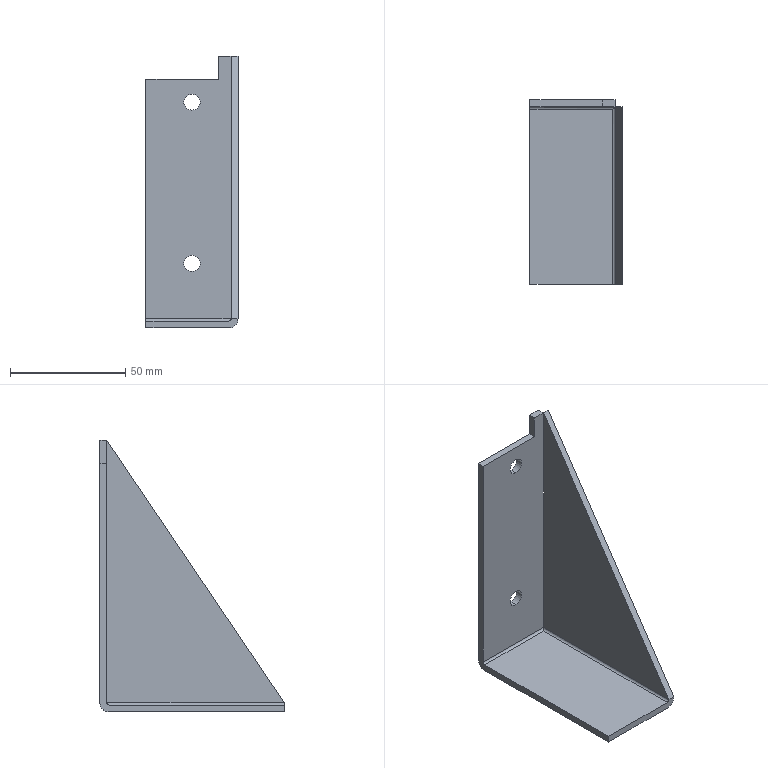Component | SolidWorks | ButtonStation-1_BracketAssembly-1_Bracket3-1 | 1 solid | 24 faces | box 40 x 80 x 118 mm | volume 34147 mm3 | plane 14 | cylinder 8 | spline 2 | commonest cylinder face diameters 7 x4 8 x2 2 x2 | material Plain Carbon Steel
STEP:
#1=CARTESIAN_POINT('',(6.299,24.685,25.846));
#2=VERTEX_POINT('',#1);
#3=CARTESIAN_POINT('',(6.299,24.685,25.571));
#4=VERTEX_POINT('',#3);
#5=CARTESIAN_POINT('',(6.299,24.685,25.709));
#6=DIRECTION('',(0.,-1.,0.));
#7=DIRECTION('',(0.,0.,1.));
#8=AXIS2_PLACEMENT_3D('',#5,#6,#7);
#9=CIRCLE('',#8,0.1378);
#10=EDGE_CURVE('',#2,#4,#9,.T.);
#11=ORIENTED_EDGE('',*,*,#10,.T.);
#12=CARTESIAN_POINT('',(6.299,24.803,25.571));
#13=VERTEX_POINT('',#12);
#14=CARTESIAN_POINT('',(6.299,24.685,25.571));
#15=DIRECTION('',(0.,1.,-0.));
#16=VECTOR('',#15,39.37);
#17=LINE('',#14,#16);
#18=EDGE_CURVE('',#4,#13,#17,.T.);
#19=ORIENTED_EDGE('',*,*,#18,.T.);
#20=CARTESIAN_POINT('',(6.299,24.803,25.846));
#21=VERTEX_POINT('',#20);
#22=CARTESIAN_POINT('',(6.299,24.803,25.709));
#23=DIRECTION('',(0.,-1.,0.));
#24=DIRECTION('',(0.,0.,1.));
#25=AXIS2_PLACEMENT_3D('',#22,#23,#24);
#26=CIRCLE('',#25,0.1378);
#27=EDGE_CURVE('',#21,#13,#26,.T.);
#28=ORIENTED_EDGE('',*,*,#27,.F.);
#29=CARTESIAN_POINT('',(6.299,24.685,25.846));
#30=DIRECTION('',(0.,1.,-0.));
#31=VECTOR('',#30,39.37);
#32=LINE('',#29,#31);
#33=EDGE_CURVE('',#2,#21,#32,.T.);
#34=ORIENTED_EDGE('',*,*,#33,.F.);
#35=EDGE_LOOP('',(#11,#19,#28,#34));
#36=FACE_OUTER_BOUND('',#35,.T.);
#37=CARTESIAN_POINT('',(6.299,24.685,25.709));
#38=DIRECTION('',(0.,1.,-0.));
#39=DIRECTION('',(0.,0.,1.));
#40=AXIS2_PLACEMENT_3D('',#37,#38,#39);
#41=CYLINDRICAL_SURFACE('',#40,0.1378);
#42=ADVANCED_FACE('',(#36),#41,.F.);
#43=CARTESIAN_POINT('',(6.299,24.685,23.091));
#44=VERTEX_POINT('',#43);
#45=CARTESIAN_POINT('',(6.299,24.685,22.815));
#46=VERTEX_POINT('',#45);
#47=CARTESIAN_POINT('',(6.299,24.685,22.953));
#48=DIRECTION('',(0.,-1.,0.));
#49=DIRECTION('',(0.,0.,1.));
#50=AXIS2_PLACEMENT_3D('',#47,#48,#49);
#51=CIRCLE('',#50,0.1378);
#52=EDGE_CURVE('',#44,#46,#51,.T.);
#53=ORIENTED_EDGE('',*,*,#52,.T.);
#54=CARTESIAN_POINT('',(6.299,24.803,22.815));
#55=VERTEX_POINT('',#54);
#56=CARTESIAN_POINT('',(6.299,24.685,22.815));
#57=DIRECTION('',(0.,1.,-0.));
#58=VECTOR('',#57,39.37);
#59=LINE('',#56,#58);
#60=EDGE_CURVE('',#46,#55,#59,.T.);
#61=ORIENTED_EDGE('',*,*,#60,.T.);
#62=CARTESIAN_POINT('',(6.299,24.803,23.091));
#63=VERTEX_POINT('',#62);
#64=CARTESIAN_POINT('',(6.299,24.803,22.953));
#65=DIRECTION('',(0.,-1.,0.));
#66=DIRECTION('',(0.,0.,1.));
#67=AXIS2_PLACEMENT_3D('',#64,#65,#66);
#68=CIRCLE('',#67,0.1378);
#69=EDGE_CURVE('',#63,#55,#68,.T.);
#70=ORIENTED_EDGE('',*,*,#69,.F.);
#71=CARTESIAN_POINT('',(6.299,24.685,23.091));
#72=DIRECTION('',(0.,1.,-0.));
#73=VECTOR('',#72,39.37);
#74=LINE('',#71,#73);
#75=EDGE_CURVE('',#44,#63,#74,.T.);
#76=ORIENTED_EDGE('',*,*,#75,.F.);
#77=EDGE_LOOP('',(#53,#61,#70,#76));
#78=FACE_OUTER_BOUND('',#77,.T.);
#79=CARTESIAN_POINT('',(6.299,24.685,22.953));
#80=DIRECTION('',(0.,1.,-0.));
#81=DIRECTION('',(0.,0.,1.));
#82=AXIS2_PLACEMENT_3D('',#79,#80,#81);
#83=CYLINDRICAL_SURFACE('',#82,0.1378);
#84=ADVANCED_FACE('',(#78),#83,.F.);
#85=CARTESIAN_POINT('',(7.087,24.682,26.496));
#86=VERTEX_POINT('',#85);
#87=CARTESIAN_POINT('',(7.087,21.654,22.008));
#88=VERTEX_POINT('',#87);
#89=CARTESIAN_POINT('',(7.087,24.682,26.496));
#90=DIRECTION('',(-0.,-0.5594,-0.8289));
#91=VECTOR('',#90,39.37);
#92=LINE('',#89,#91);
#93=EDGE_CURVE('',#86,#88,#92,.T.);
#94=ORIENTED_EDGE('',*,*,#93,.T.);
#95=CARTESIAN_POINT('',(7.087,24.682,22.008));
#96=VERTEX_POINT('',#95);
#97=CARTESIAN_POINT('',(7.087,24.685,22.008));
#98=DIRECTION('',(0.,1.,0.));
#99=VECTOR('',#98,39.37);
#100=LINE('',#97,#99);
#101=EDGE_CURVE('',#88,#96,#100,.T.);
#102=ORIENTED_EDGE('',*,*,#101,.T.);
#103=CARTESIAN_POINT('',(7.087,24.682,21.969));
#104=DIRECTION('',(0.,0.,1.));
#105=VECTOR('',#104,39.37);
#106=LINE('',#103,#105);
#107=EDGE_CURVE('',#96,#86,#106,.T.);
#108=ORIENTED_EDGE('',*,*,#107,.T.);
#109=EDGE_LOOP('',(#94,#102,#108));
#110=FACE_OUTER_BOUND('',#109,.T.);
#111=CARTESIAN_POINT('',(7.087,24.685,21.969));
#112=DIRECTION('',(1.,0.,-0.));
#113=DIRECTION('',(-0.,0.,-1.));
#114=AXIS2_PLACEMENT_3D('',#111,#112,#113);
#115=PLANE('',#114);
#116=ADVANCED_FACE('',(#110),#115,.T.);
#117=ORIENTED_EDGE('',*,*,#101,.F.);
#118=CARTESIAN_POINT('',(6.929,21.654,21.85));
#119=VERTEX_POINT('',#118);
#120=CARTESIAN_POINT('',(6.929,21.654,22.008));
#121=DIRECTION('',(0.,1.,0.));
#122=DIRECTION('',(0.,0.,1.));
#123=AXIS2_PLACEMENT_3D('',#120,#121,#122);
#124=CIRCLE('',#123,0.1575);
#125=EDGE_CURVE('',#88,#119,#124,.T.);
#126=ORIENTED_EDGE('',*,*,#125,.T.);
#127=CARTESIAN_POINT('',(6.929,24.646,21.85));
#128=VERTEX_POINT('',#127);
#129=CARTESIAN_POINT('',(6.929,24.682,21.85));
#130=DIRECTION('',(0.,1.,0.));
#131=VECTOR('',#130,39.37);
#132=LINE('',#129,#131);
#133=EDGE_CURVE('',#119,#128,#132,.T.);
#134=ORIENTED_EDGE('',*,*,#133,.T.);
#135=CARTESIAN_POINT('',(6.929,24.646,21.85));
#136=CARTESIAN_POINT('',(6.95,24.649,21.85));
#137=CARTESIAN_POINT('',(6.97,24.652,21.854));
#138=CARTESIAN_POINT('',(6.999,24.656,21.866));
#139=CARTESIAN_POINT('',(7.008,24.658,21.871));
#140=CARTESIAN_POINT('',(7.025,24.661,21.883));
#141=CARTESIAN_POINT('',(7.033,24.662,21.889));
#142=CARTESIAN_POINT('',(7.048,24.665,21.904));
#143=CARTESIAN_POINT('',(7.054,24.667,21.912));
#144=CARTESIAN_POINT('',(7.066,24.67,21.929));
#145=CARTESIAN_POINT('',(7.071,24.672,21.938));
#146=CARTESIAN_POINT('',(7.079,24.675,21.957));
#147=CARTESIAN_POINT('',(7.082,24.676,21.967));
#148=CARTESIAN_POINT('',(7.086,24.679,21.987));
#149=CARTESIAN_POINT('',(7.087,24.681,21.997));
#150=CARTESIAN_POINT('',(7.087,24.682,22.008));
#151=B_SPLINE_CURVE_WITH_KNOTS('',3,(#135,#136,#137,#138,#139,#140,#141,#142,#143,#144,#145,#146,#147,#148,#149,#150),.UNSPECIFIED.,.F.,.F.,(4,2,2,2,2,2,2,4),(0.,0.001573,0.00236,0.003146,0.003933,0.00472,0.005506,0.006293),.UNSPECIFIED.);
#152=EDGE_CURVE('',#128,#96,#151,.T.);
#153=ORIENTED_EDGE('',*,*,#152,.T.);
#154=EDGE_LOOP('',(#117,#126,#134,#153));
#155=FACE_OUTER_BOUND('',#154,.T.);
#156=CARTESIAN_POINT('',(6.929,24.682,22.008));
#157=DIRECTION('',(0.,1.,0.));
#158=DIRECTION('',(0.,0.,1.));
#159=AXIS2_PLACEMENT_3D('',#156,#157,#158);
#160=CYLINDRICAL_SURFACE('',#159,0.1575);
#161=ADVANCED_FACE('',(#155),#160,.T.);
#162=CARTESIAN_POINT('',(6.969,24.682,26.496));
#163=VERTEX_POINT('',#162);
#164=CARTESIAN_POINT('',(7.087,24.682,26.496));
#165=DIRECTION('',(1.,0.,-0.));
#166=VECTOR('',#165,39.37);
#167=LINE('',#164,#166);
#168=EDGE_CURVE('',#163,#86,#167,.T.);
#169=ORIENTED_EDGE('',*,*,#168,.F.);
#170=CARTESIAN_POINT('',(6.969,21.654,22.008));
#171=VERTEX_POINT('',#170);
#172=CARTESIAN_POINT('',(6.969,21.654,22.008));
#173=DIRECTION('',(0.,0.5594,0.8289));
#174=VECTOR('',#173,39.37);
#175=LINE('',#172,#174);
#176=EDGE_CURVE('',#171,#163,#175,.T.);
#177=ORIENTED_EDGE('',*,*,#176,.F.);
#178=CARTESIAN_POINT('',(7.087,21.654,22.008));
#179=DIRECTION('',(-1.,-0.,0.));
#180=VECTOR('',#179,39.37);
#181=LINE('',#178,#180);
#182=EDGE_CURVE('',#88,#171,#181,.T.);
#183=ORIENTED_EDGE('',*,*,#182,.F.);
#184=ORIENTED_EDGE('',*,*,#93,.F.);
#185=EDGE_LOOP('',(#169,#177,#183,#184));
#186=FACE_OUTER_BOUND('',#185,.T.);
#187=CARTESIAN_POINT('',(7.087,21.654,22.008));
#188=DIRECTION('',(-0.,0.8289,-0.5594));
#189=DIRECTION('',(0.,0.5594,0.8289));
#190=AXIS2_PLACEMENT_3D('',#187,#188,#189);
#191=PLANE('',#190);
#192=ADVANCED_FACE('',(#186),#191,.F.);
#193=ORIENTED_EDGE('',*,*,#168,.T.);
#194=ORIENTED_EDGE('',*,*,#107,.F.);
#195=CARTESIAN_POINT('',(6.969,24.682,22.008));
#196=VERTEX_POINT('',#195);
#197=CARTESIAN_POINT('',(6.969,24.682,22.008));
#198=DIRECTION('',(1.,0.,0.));
#199=VECTOR('',#198,39.37);
#200=LINE('',#197,#199);
#201=EDGE_CURVE('',#196,#96,#200,.T.);
#202=ORIENTED_EDGE('',*,*,#201,.F.);
#203=CARTESIAN_POINT('',(6.969,24.682,21.969));
#204=DIRECTION('',(0.,0.,-1.));
#205=VECTOR('',#204,39.37);
#206=LINE('',#203,#205);
#207=EDGE_CURVE('',#163,#196,#206,.T.);
#208=ORIENTED_EDGE('',*,*,#207,.F.);
#209=EDGE_LOOP('',(#193,#194,#202,#208));
#210=FACE_OUTER_BOUND('',#209,.T.);
#211=CARTESIAN_POINT('',(6.969,24.682,21.969));
#212=DIRECTION('',(0.,-1.,0.));
#213=DIRECTION('',(0.,0.,-1.));
#214=AXIS2_PLACEMENT_3D('',#211,#212,#213);
#215=PLANE('',#214);
#216=ADVANCED_FACE('',(#210),#215,.F.);
#217=CARTESIAN_POINT('',(6.929,21.654,21.969));
#218=VERTEX_POINT('',#217);
#219=CARTESIAN_POINT('',(6.929,21.654,22.008));
#220=DIRECTION('',(0.,1.,0.));
#221=DIRECTION('',(0.,0.,1.));
#222=AXIS2_PLACEMENT_3D('',#219,#220,#221);
#223=CIRCLE('',#222,0.03937);
#224=EDGE_CURVE('',#171,#218,#223,.T.);
#225=ORIENTED_EDGE('',*,*,#224,.T.);
#226=CARTESIAN_POINT('',(5.512,21.654,21.969));
#227=VERTEX_POINT('',#226);
#228=CARTESIAN_POINT('',(5.512,21.654,21.969));
#229=DIRECTION('',(1.,0.,0.));
#230=VECTOR('',#229,39.37);
#231=LINE('',#228,#230);
#232=EDGE_CURVE('',#227,#218,#231,.T.);
#233=ORIENTED_EDGE('',*,*,#232,.F.);
#234=CARTESIAN_POINT('',(5.512,21.654,21.85));
#235=VERTEX_POINT('',#234);
#236=CARTESIAN_POINT('',(5.512,21.654,21.969));
#237=DIRECTION('',(0.,0.,1.));
#238=VECTOR('',#237,39.37);
#239=LINE('',#236,#238);
#240=EDGE_CURVE('',#235,#227,#239,.T.);
#241=ORIENTED_EDGE('',*,*,#240,.F.);
#242=CARTESIAN_POINT('',(5.512,21.654,21.85));
#243=DIRECTION('',(-1.,0.,0.));
#244=VECTOR('',#243,39.37);
#245=LINE('',#242,#244);
#246=EDGE_CURVE('',#119,#235,#245,.T.);
#247=ORIENTED_EDGE('',*,*,#246,.F.);
#248=ORIENTED_EDGE('',*,*,#125,.F.);
#249=ORIENTED_EDGE('',*,*,#182,.T.);
#250=EDGE_LOOP('',(#225,#233,#241,#247,#248,#249));
#251=FACE_OUTER_BOUND('',#250,.T.);
#252=CARTESIAN_POINT('',(6.929,21.654,22.008));
#253=DIRECTION('',(0.,-1.,0.));
#254=DIRECTION('',(0.,0.,-1.));
#255=AXIS2_PLACEMENT_3D('',#252,#253,#254);
#256=PLANE('',#255);
#257=ADVANCED_FACE('',(#251),#256,.T.);
#258=ORIENTED_EDGE('',*,*,#201,.T.);
#259=ORIENTED_EDGE('',*,*,#152,.F.);
#260=CARTESIAN_POINT('',(6.929,24.646,21.969));
#261=VERTEX_POINT('',#260);
#262=CARTESIAN_POINT('',(6.929,24.646,21.909));
#263=DIRECTION('',(0.,0.,-1.));
#264=VECTOR('',#263,39.37);
#265=LINE('',#262,#264);
#266=EDGE_CURVE('',#261,#128,#265,.T.);
#267=ORIENTED_EDGE('',*,*,#266,.F.);
#268=CARTESIAN_POINT('',(6.969,24.682,22.008));
#269=CARTESIAN_POINT('',(6.969,24.679,22.003));
#270=CARTESIAN_POINT('',(6.967,24.676,21.998));
#271=CARTESIAN_POINT('',(6.964,24.67,21.988));
#272=CARTESIAN_POINT('',(6.961,24.667,21.984));
#273=CARTESIAN_POINT('',(6.953,24.661,21.976));
#274=CARTESIAN_POINT('',(6.949,24.658,21.974));
#275=CARTESIAN_POINT('',(6.939,24.652,21.97));
#276=CARTESIAN_POINT('',(6.934,24.649,21.969));
#277=CARTESIAN_POINT('',(6.929,24.646,21.969));
#278=B_SPLINE_CURVE_WITH_KNOTS('',3,(#268,#269,#270,#271,#272,#273,#274,#275,#276,#277),.UNSPECIFIED.,.F.,.F.,(4,2,2,2,4),(0.,0.0004525,0.000905,0.001358,0.00181),.UNSPECIFIED.);
#279=EDGE_CURVE('',#196,#261,#278,.T.);
#280=ORIENTED_EDGE('',*,*,#279,.F.);
#281=EDGE_LOOP('',(#258,#259,#267,#280));
#282=FACE_OUTER_BOUND('',#281,.T.);
#283=CARTESIAN_POINT('',(7.088,24.682,22.008));
#284=CARTESIAN_POINT('',(7.088,24.679,21.987));
#285=CARTESIAN_POINT('',(7.084,24.676,21.966));
#286=CARTESIAN_POINT('',(7.068,24.67,21.928));
#287=CARTESIAN_POINT('',(7.056,24.667,21.91));
#288=CARTESIAN_POINT('',(7.027,24.661,21.881));
#289=CARTESIAN_POINT('',(7.009,24.658,21.869));
#290=CARTESIAN_POINT('',(6.971,24.652,21.853));
#291=CARTESIAN_POINT('',(6.95,24.649,21.849));
#292=CARTESIAN_POINT('',(6.929,24.646,21.849));
#293=CARTESIAN_POINT('',(7.087,24.682,22.008));
#294=CARTESIAN_POINT('',(7.087,24.679,21.987));
#295=CARTESIAN_POINT('',(7.083,24.676,21.967));
#296=CARTESIAN_POINT('',(7.067,24.67,21.929));
#297=CARTESIAN_POINT('',(7.055,24.667,21.911));
#298=CARTESIAN_POINT('',(7.026,24.661,21.882));
#299=CARTESIAN_POINT('',(7.008,24.658,21.87));
#300=CARTESIAN_POINT('',(6.97,24.652,21.854));
#301=CARTESIAN_POINT('',(6.95,24.649,21.85));
#302=CARTESIAN_POINT('',(6.929,24.646,21.85));
#303=CARTESIAN_POINT('',(6.969,24.682,22.008));
#304=CARTESIAN_POINT('',(6.969,24.679,22.003));
#305=CARTESIAN_POINT('',(6.967,24.676,21.998));
#306=CARTESIAN_POINT('',(6.964,24.67,21.988));
#307=CARTESIAN_POINT('',(6.961,24.667,21.984));
#308=CARTESIAN_POINT('',(6.953,24.661,21.976));
#309=CARTESIAN_POINT('',(6.949,24.658,21.973));
#310=CARTESIAN_POINT('',(6.939,24.652,21.97));
#311=CARTESIAN_POINT('',(6.934,24.649,21.969));
#312=CARTESIAN_POINT('',(6.929,24.646,21.969));
#313=CARTESIAN_POINT('',(6.967,24.682,22.008));
#314=CARTESIAN_POINT('',(6.967,24.679,22.003));
#315=CARTESIAN_POINT('',(6.966,24.676,21.998));
#316=CARTESIAN_POINT('',(6.962,24.67,21.989));
#317=CARTESIAN_POINT('',(6.96,24.667,21.984));
#318=CARTESIAN_POINT('',(6.953,24.661,21.977));
#319=CARTESIAN_POINT('',(6.948,24.658,21.975));
#320=CARTESIAN_POINT('',(6.939,24.652,21.971));
#321=CARTESIAN_POINT('',(6.934,24.649,21.97));
#322=CARTESIAN_POINT('',(6.929,24.646,21.97));
#323=B_SPLINE_SURFACE_WITH_KNOTS('',1,3,((#283,#284,#285,#286,#287,#288,#289,#290,#291,#292),(#293,#294,#295,#296,#297,#298,#299,#300,#301,#302),(#303,#304,#305,#306,#307,#308,#309,#310,#311,#312),(#313,#314,#315,#316,#317,#318,#319,#320,#321,#322)),.UNSPECIFIED.,.F.,.F.,.F.,(2,1,1,2),(4,2,2,2,4),(-0.01,0.,1.,1.01),(0.,0.25,0.5,0.75,1.),.UNSPECIFIED.);
#324=ADVANCED_FACE('',(#282),#323,.F.);
#325=ORIENTED_EDGE('',*,*,#246,.T.);
#326=CARTESIAN_POINT('',(5.512,24.646,21.85));
#327=VERTEX_POINT('',#326);
#328=CARTESIAN_POINT('',(5.512,24.685,21.85));
#329=DIRECTION('',(0.,1.,0.));
#330=VECTOR('',#329,39.37);
#331=LINE('',#328,#330);
#332=EDGE_CURVE('',#235,#327,#331,.T.);
#333=ORIENTED_EDGE('',*,*,#332,.T.);
#334=CARTESIAN_POINT('',(5.512,24.646,21.85));
#335=DIRECTION('',(1.,0.,0.));
#336=VECTOR('',#335,39.37);
#337=LINE('',#334,#336);
#338=EDGE_CURVE('',#327,#128,#337,.T.);
#339=ORIENTED_EDGE('',*,*,#338,.T.);
#340=ORIENTED_EDGE('',*,*,#133,.F.);
#341=EDGE_LOOP('',(#325,#333,#339,#340));
#342=FACE_OUTER_BOUND('',#341,.T.);
#343=CARTESIAN_POINT('',(5.512,24.685,21.85));
#344=DIRECTION('',(0.,0.,-1.));
#345=DIRECTION('',(-1.,0.,0.));
#346=AXIS2_PLACEMENT_3D('',#343,#344,#345);
#347=PLANE('',#346);
#348=ADVANCED_FACE('',(#342),#347,.T.);
#349=ORIENTED_EDGE('',*,*,#207,.T.);
#350=CARTESIAN_POINT('',(6.969,24.685,22.008));
#351=DIRECTION('',(0.,1.,0.));
#352=VECTOR('',#351,39.37);
#353=LINE('',#350,#352);
#354=EDGE_CURVE('',#171,#196,#353,.T.);
#355=ORIENTED_EDGE('',*,*,#354,.F.);
#356=ORIENTED_EDGE('',*,*,#176,.T.);
#357=EDGE_LOOP('',(#349,#355,#356));
#358=FACE_OUTER_BOUND('',#357,.T.);
#359=CARTESIAN_POINT('',(6.969,24.685,21.969));
#360=DIRECTION('',(1.,0.,-0.));
#361=DIRECTION('',(-0.,0.,-1.));
#362=AXIS2_PLACEMENT_3D('',#359,#360,#361);
#363=PLANE('',#362);
#364=ADVANCED_FACE('',(#358),#363,.F.);
#365=ORIENTED_EDGE('',*,*,#224,.F.);
#366=ORIENTED_EDGE('',*,*,#354,.T.);
#367=ORIENTED_EDGE('',*,*,#279,.T.);
#368=CARTESIAN_POINT('',(6.929,24.682,21.969));
#369=DIRECTION('',(0.,1.,0.));
#370=VECTOR('',#369,39.37);
#371=LINE('',#368,#370);
#372=EDGE_CURVE('',#218,#261,#371,.T.);
#373=ORIENTED_EDGE('',*,*,#372,.F.);
#374=EDGE_LOOP('',(#365,#366,#367,#373));
#375=FACE_OUTER_BOUND('',#374,.T.);
#376=CARTESIAN_POINT('',(6.929,24.682,22.008));
#377=DIRECTION('',(0.,1.,0.));
#378=DIRECTION('',(0.,0.,1.));
#379=AXIS2_PLACEMENT_3D('',#376,#377,#378);
#380=CYLINDRICAL_SURFACE('',#379,0.03937);
#381=ADVANCED_FACE('',(#375),#380,.F.);
#382=CARTESIAN_POINT('',(6.966,24.685,22.008));
#383=VERTEX_POINT('',#382);
#384=CARTESIAN_POINT('',(6.929,24.646,21.969));
#385=CARTESIAN_POINT('',(6.932,24.651,21.969));
#386=CARTESIAN_POINT('',(6.935,24.656,21.97));
#387=CARTESIAN_POINT('',(6.941,24.665,21.973));
#388=CARTESIAN_POINT('',(6.944,24.67,21.976));
#389=CARTESIAN_POINT('',(6.95,24.677,21.984));
#390=CARTESIAN_POINT('',(6.953,24.68,21.988));
#391=CARTESIAN_POINT('',(6.96,24.684,21.998));
#392=CARTESIAN_POINT('',(6.963,24.685,22.003));
#393=CARTESIAN_POINT('',(6.966,24.685,22.008));
#394=B_SPLINE_CURVE_WITH_KNOTS('',3,(#384,#385,#386,#387,#388,#389,#390,#391,#392,#393),.UNSPECIFIED.,.F.,.F.,(4,2,2,2,4),(0.,0.0004525,0.000905,0.001358,0.00181),.UNSPECIFIED.);
#395=EDGE_CURVE('',#261,#383,#394,.T.);
#396=ORIENTED_EDGE('',*,*,#395,.F.);
#397=ORIENTED_EDGE('',*,*,#266,.T.);
#398=CARTESIAN_POINT('',(6.966,24.803,22.008));
#399=VERTEX_POINT('',#398);
#400=CARTESIAN_POINT('',(6.966,24.803,22.008));
#401=CARTESIAN_POINT('',(6.963,24.803,21.987));
#402=CARTESIAN_POINT('',(6.96,24.799,21.967));
#403=CARTESIAN_POINT('',(6.955,24.787,21.938));
#404=CARTESIAN_POINT('',(6.954,24.782,21.929));
#405=CARTESIAN_POINT('',(6.951,24.771,21.912));
#406=CARTESIAN_POINT('',(6.949,24.764,21.904));
#407=CARTESIAN_POINT('',(6.946,24.75,21.889));
#408=CARTESIAN_POINT('',(6.944,24.742,21.883));
#409=CARTESIAN_POINT('',(6.941,24.725,21.871));
#410=CARTESIAN_POINT('',(6.94,24.716,21.866));
#411=CARTESIAN_POINT('',(6.937,24.697,21.858));
#412=CARTESIAN_POINT('',(6.935,24.687,21.855));
#413=CARTESIAN_POINT('',(6.932,24.666,21.851));
#414=CARTESIAN_POINT('',(6.931,24.656,21.85));
#415=CARTESIAN_POINT('',(6.929,24.646,21.85));
#416=B_SPLINE_CURVE_WITH_KNOTS('',3,(#400,#401,#402,#403,#404,#405,#406,#407,#408,#409,#410,#411,#412,#413,#414,#415),.UNSPECIFIED.,.F.,.F.,(4,2,2,2,2,2,2,4),(0.,0.001573,0.00236,0.003146,0.003933,0.00472,0.005506,0.006293),.UNSPECIFIED.);
#417=EDGE_CURVE('',#399,#128,#416,.T.);
#418=ORIENTED_EDGE('',*,*,#417,.F.);
#419=CARTESIAN_POINT('',(6.966,24.744,22.008));
#420=DIRECTION('',(0.,1.,0.));
#421=VECTOR('',#420,39.37);
#422=LINE('',#419,#421);
#423=EDGE_CURVE('',#383,#399,#422,.T.);
#424=ORIENTED_EDGE('',*,*,#423,.F.);
#425=EDGE_LOOP('',(#396,#397,#418,#424));
#426=FACE_OUTER_BOUND('',#425,.T.);
#427=CARTESIAN_POINT('',(6.929,24.646,21.849));
#428=CARTESIAN_POINT('',(6.932,24.666,21.849));
#429=CARTESIAN_POINT('',(6.935,24.687,21.853));
#430=CARTESIAN_POINT('',(6.941,24.726,21.869));
#431=CARTESIAN_POINT('',(6.944,24.743,21.881));
#432=CARTESIAN_POINT('',(6.95,24.773,21.91));
#433=CARTESIAN_POINT('',(6.954,24.784,21.928));
#434=CARTESIAN_POINT('',(6.96,24.8,21.966));
#435=CARTESIAN_POINT('',(6.963,24.804,21.987));
#436=CARTESIAN_POINT('',(6.966,24.804,22.008));
#437=CARTESIAN_POINT('',(6.929,24.646,21.85));
#438=CARTESIAN_POINT('',(6.932,24.666,21.85));
#439=CARTESIAN_POINT('',(6.935,24.687,21.854));
#440=CARTESIAN_POINT('',(6.941,24.725,21.87));
#441=CARTESIAN_POINT('',(6.944,24.742,21.882));
#442=CARTESIAN_POINT('',(6.95,24.772,21.911));
#443=CARTESIAN_POINT('',(6.954,24.783,21.929));
#444=CARTESIAN_POINT('',(6.96,24.799,21.967));
#445=CARTESIAN_POINT('',(6.963,24.803,21.987));
#446=CARTESIAN_POINT('',(6.966,24.803,22.008));
#447=CARTESIAN_POINT('',(6.929,24.646,21.969));
#448=CARTESIAN_POINT('',(6.932,24.651,21.969));
#449=CARTESIAN_POINT('',(6.935,24.656,21.97));
#450=CARTESIAN_POINT('',(6.941,24.665,21.973));
#451=CARTESIAN_POINT('',(6.944,24.67,21.976));
#452=CARTESIAN_POINT('',(6.95,24.677,21.984));
#453=CARTESIAN_POINT('',(6.954,24.68,21.988));
#454=CARTESIAN_POINT('',(6.96,24.684,21.998));
#455=CARTESIAN_POINT('',(6.963,24.685,22.003));
#456=CARTESIAN_POINT('',(6.966,24.685,22.008));
#457=CARTESIAN_POINT('',(6.929,24.646,21.97));
#458=CARTESIAN_POINT('',(6.932,24.651,21.97));
#459=CARTESIAN_POINT('',(6.935,24.656,21.971));
#460=CARTESIAN_POINT('',(6.941,24.665,21.975));
#461=CARTESIAN_POINT('',(6.944,24.669,21.977));
#462=CARTESIAN_POINT('',(6.95,24.676,21.984));
#463=CARTESIAN_POINT('',(6.954,24.679,21.989));
#464=CARTESIAN_POINT('',(6.96,24.683,21.998));
#465=CARTESIAN_POINT('',(6.963,24.684,22.003));
#466=CARTESIAN_POINT('',(6.966,24.684,22.008));
#467=B_SPLINE_SURFACE_WITH_KNOTS('',1,3,((#427,#428,#429,#430,#431,#432,#433,#434,#435,#436),(#437,#438,#439,#440,#441,#442,#443,#444,#445,#446),(#447,#448,#449,#450,#451,#452,#453,#454,#455,#456),(#457,#458,#459,#460,#461,#462,#463,#464,#465,#466)),.UNSPECIFIED.,.F.,.F.,.F.,(2,1,1,2),(4,2,2,2,4),(-0.01,0.,1.,1.01),(0.,0.25,0.5,0.75,1.),.UNSPECIFIED.);
#468=ADVANCED_FACE('',(#426),#467,.F.);
#469=CARTESIAN_POINT('',(5.512,24.685,22.008));
#470=VERTEX_POINT('',#469);
#471=CARTESIAN_POINT('',(5.512,24.685,26.102));
#472=VERTEX_POINT('',#471);
#473=CARTESIAN_POINT('',(5.512,24.685,21.969));
#474=DIRECTION('',(0.,0.,1.));
#475=VECTOR('',#474,39.37);
#476=LINE('',#473,#475);
#477=EDGE_CURVE('',#470,#472,#476,.T.);
#478=ORIENTED_EDGE('',*,*,#477,.T.);
#479=CARTESIAN_POINT('',(5.512,24.803,26.102));
#480=VERTEX_POINT('',#479);
#481=CARTESIAN_POINT('',(5.512,21.654,26.102));
#482=DIRECTION('',(0.,1.,0.));
#483=VECTOR('',#482,39.37);
#484=LINE('',#481,#483);
#485=EDGE_CURVE('',#472,#480,#484,.T.);
#486=ORIENTED_EDGE('',*,*,#485,.T.);
#487=CARTESIAN_POINT('',(5.512,24.803,22.008));
#488=VERTEX_POINT('',#487);
#489=CARTESIAN_POINT('',(5.512,24.803,21.969));
#490=DIRECTION('',(0.,0.,1.));
#491=VECTOR('',#490,39.37);
#492=LINE('',#489,#491);
#493=EDGE_CURVE('',#488,#480,#492,.T.);
#494=ORIENTED_EDGE('',*,*,#493,.F.);
#495=CARTESIAN_POINT('',(5.512,24.646,22.008));
#496=DIRECTION('',(1.,0.,0.));
#497=DIRECTION('',(0.,0.,1.));
#498=AXIS2_PLACEMENT_3D('',#495,#496,#497);
#499=CIRCLE('',#498,0.1575);
#500=EDGE_CURVE('',#327,#488,#499,.T.);
#501=ORIENTED_EDGE('',*,*,#500,.F.);
#502=ORIENTED_EDGE('',*,*,#332,.F.);
#503=ORIENTED_EDGE('',*,*,#240,.T.);
#504=CARTESIAN_POINT('',(5.512,24.646,21.969));
#505=VERTEX_POINT('',#504);
#506=CARTESIAN_POINT('',(5.512,21.654,21.969));
#507=DIRECTION('',(0.,-1.,0.));
#508=VECTOR('',#507,39.37);
#509=LINE('',#506,#508);
#510=EDGE_CURVE('',#505,#227,#509,.T.);
#511=ORIENTED_EDGE('',*,*,#510,.F.);
#512=CARTESIAN_POINT('',(5.512,24.646,22.008));
#513=DIRECTION('',(1.,0.,0.));
#514=DIRECTION('',(0.,0.,1.));
#515=AXIS2_PLACEMENT_3D('',#512,#513,#514);
#516=CIRCLE('',#515,0.03937);
#517=EDGE_CURVE('',#505,#470,#516,.T.);
#518=ORIENTED_EDGE('',*,*,#517,.T.);
#519=EDGE_LOOP('',(#478,#486,#494,#501,#502,#503,#511,#518));
#520=FACE_OUTER_BOUND('',#519,.T.);
#521=CARTESIAN_POINT('',(5.512,21.654,21.969));
#522=DIRECTION('',(1.,0.,0.));
#523=DIRECTION('',(0.,0.,-1.));
#524=AXIS2_PLACEMENT_3D('',#521,#522,#523);
#525=PLANE('',#524);
#526=ADVANCED_FACE('',(#520),#525,.F.);
#527=CARTESIAN_POINT('',(5.512,24.803,22.008));
#528=DIRECTION('',(1.,0.,0.));
#529=VECTOR('',#528,39.37);
#530=LINE('',#527,#529);
#531=EDGE_CURVE('',#488,#399,#530,.T.);
#532=ORIENTED_EDGE('',*,*,#531,.T.);
#533=ORIENTED_EDGE('',*,*,#417,.T.);
#534=ORIENTED_EDGE('',*,*,#338,.F.);
#535=ORIENTED_EDGE('',*,*,#500,.T.);
#536=EDGE_LOOP('',(#532,#533,#534,#535));
#537=FACE_OUTER_BOUND('',#536,.T.);
#538=CARTESIAN_POINT('',(5.512,24.646,22.008));
#539=DIRECTION('',(-1.,0.,0.));
#540=DIRECTION('',(0.,0.,1.));
#541=AXIS2_PLACEMENT_3D('',#538,#539,#540);
#542=CYLINDRICAL_SURFACE('',#541,0.1575);
#543=ADVANCED_FACE('',(#537),#542,.T.);
#544=CARTESIAN_POINT('',(5.512,24.646,21.969));
#545=DIRECTION('',(1.,0.,0.));
#546=VECTOR('',#545,39.37);
#547=LINE('',#544,#546);
#548=EDGE_CURVE('',#505,#261,#547,.T.);
#549=ORIENTED_EDGE('',*,*,#548,.F.);
#550=ORIENTED_EDGE('',*,*,#510,.T.);
#551=ORIENTED_EDGE('',*,*,#232,.T.);
#552=ORIENTED_EDGE('',*,*,#372,.T.);
#553=EDGE_LOOP('',(#549,#550,#551,#552));
#554=FACE_OUTER_BOUND('',#553,.T.);
#555=CARTESIAN_POINT('',(5.512,24.685,21.969));
#556=DIRECTION('',(0.,0.,-1.));
#557=DIRECTION('',(-1.,0.,0.));
#558=AXIS2_PLACEMENT_3D('',#555,#556,#557);
#559=PLANE('',#558);
#560=ADVANCED_FACE('',(#554),#559,.F.);
#561=ORIENTED_EDGE('',*,*,#423,.T.);
#562=CARTESIAN_POINT('',(6.966,24.803,26.496));
#563=VERTEX_POINT('',#562);
#564=CARTESIAN_POINT('',(6.966,24.803,21.969));
#565=DIRECTION('',(0.,0.,1.));
#566=VECTOR('',#565,39.37);
#567=LINE('',#564,#566);
#568=EDGE_CURVE('',#399,#563,#567,.T.);
#569=ORIENTED_EDGE('',*,*,#568,.T.);
#570=CARTESIAN_POINT('',(6.966,24.685,26.496));
#571=VERTEX_POINT('',#570);
#572=CARTESIAN_POINT('',(6.966,24.685,26.496));
#573=DIRECTION('',(0.,-1.,0.));
#574=VECTOR('',#573,39.37);
#575=LINE('',#572,#574);
#576=EDGE_CURVE('',#563,#571,#575,.T.);
#577=ORIENTED_EDGE('',*,*,#576,.T.);
#578=CARTESIAN_POINT('',(6.966,24.685,21.969));
#579=DIRECTION('',(0.,0.,-1.));
#580=VECTOR('',#579,39.37);
#581=LINE('',#578,#580);
#582=EDGE_CURVE('',#571,#383,#581,.T.);
#583=ORIENTED_EDGE('',*,*,#582,.T.);
#584=EDGE_LOOP('',(#561,#569,#577,#583));
#585=FACE_OUTER_BOUND('',#584,.T.);
#586=CARTESIAN_POINT('',(6.966,24.685,21.969));
#587=DIRECTION('',(1.,0.,0.));
#588=DIRECTION('',(0.,0.,-1.));
#589=AXIS2_PLACEMENT_3D('',#586,#587,#588);
#590=PLANE('',#589);
#591=ADVANCED_FACE('',(#585),#590,.T.);
#592=ORIENTED_EDGE('',*,*,#395,.T.);
#593=CARTESIAN_POINT('',(5.512,24.685,22.008));
#594=DIRECTION('',(1.,0.,0.));
#595=VECTOR('',#594,39.37);
#596=LINE('',#593,#595);
#597=EDGE_CURVE('',#470,#383,#596,.T.);
#598=ORIENTED_EDGE('',*,*,#597,.F.);
#599=ORIENTED_EDGE('',*,*,#517,.F.);
#600=ORIENTED_EDGE('',*,*,#548,.T.);
#601=EDGE_LOOP('',(#592,#598,#599,#600));
#602=FACE_OUTER_BOUND('',#601,.T.);
#603=CARTESIAN_POINT('',(5.512,24.646,22.008));
#604=DIRECTION('',(-1.,0.,0.));
#605=DIRECTION('',(0.,0.,1.));
#606=AXIS2_PLACEMENT_3D('',#603,#604,#605);
#607=CYLINDRICAL_SURFACE('',#606,0.03937);
#608=ADVANCED_FACE('',(#602),#607,.F.);
#609=CARTESIAN_POINT('',(6.752,24.803,26.496));
#610=VERTEX_POINT('',#609);
#611=CARTESIAN_POINT('',(6.752,24.803,26.102));
#612=VERTEX_POINT('',#611);
#613=CARTESIAN_POINT('',(6.752,24.803,21.969));
#614=DIRECTION('',(0.,-0.,-1.));
#615=VECTOR('',#614,39.37);
#616=LINE('',#613,#615);
#617=EDGE_CURVE('',#610,#612,#616,.T.);
#618=ORIENTED_EDGE('',*,*,#617,.F.);
#619=CARTESIAN_POINT('',(5.512,24.803,26.496));
#620=DIRECTION('',(1.,0.,0.));
#621=VECTOR('',#620,39.37);
#622=LINE('',#619,#621);
#623=EDGE_CURVE('',#610,#563,#622,.T.);
#624=ORIENTED_EDGE('',*,*,#623,.T.);
#625=ORIENTED_EDGE('',*,*,#568,.F.);
#626=ORIENTED_EDGE('',*,*,#531,.F.);
#627=ORIENTED_EDGE('',*,*,#493,.T.);
#628=CARTESIAN_POINT('',(5.512,24.803,26.102));
#629=DIRECTION('',(-1.,0.,0.));
#630=VECTOR('',#629,39.37);
#631=LINE('',#628,#630);
#632=EDGE_CURVE('',#612,#480,#631,.T.);
#633=ORIENTED_EDGE('',*,*,#632,.F.);
#634=EDGE_LOOP('',(#618,#624,#625,#626,#627,#633));
#635=FACE_OUTER_BOUND('',#634,.T.);
#636=ORIENTED_EDGE('',*,*,#27,.T.);
#637=CARTESIAN_POINT('',(6.299,24.803,25.709));
#638=DIRECTION('',(0.,-1.,0.));
#639=DIRECTION('',(0.,0.,1.));
#640=AXIS2_PLACEMENT_3D('',#637,#638,#639);
#641=CIRCLE('',#640,0.1378);
#642=EDGE_CURVE('',#13,#21,#641,.T.);
#643=ORIENTED_EDGE('',*,*,#642,.T.);
#644=EDGE_LOOP('',(#636,#643));
#645=FACE_BOUND('',#644,.T.);
#646=ORIENTED_EDGE('',*,*,#69,.T.);
#647=CARTESIAN_POINT('',(6.299,24.803,22.953));
#648=DIRECTION('',(0.,-1.,0.));
#649=DIRECTION('',(0.,0.,1.));
#650=AXIS2_PLACEMENT_3D('',#647,#648,#649);
#651=CIRCLE('',#650,0.1378);
#652=EDGE_CURVE('',#55,#63,#651,.T.);
#653=ORIENTED_EDGE('',*,*,#652,.T.);
#654=EDGE_LOOP('',(#646,#653));
#655=FACE_BOUND('',#654,.T.);
#656=CARTESIAN_POINT('',(5.512,24.803,21.969));
#657=DIRECTION('',(0.,1.,-0.));
#658=DIRECTION('',(0.,0.,1.));
#659=AXIS2_PLACEMENT_3D('',#656,#657,#658);
#660=PLANE('',#659);
#661=ADVANCED_FACE('',(#635,#645,#655),#660,.T.);
#662=CARTESIAN_POINT('',(6.752,24.685,26.496));
#663=VERTEX_POINT('',#662);
#664=CARTESIAN_POINT('',(6.752,24.685,26.102));
#665=VERTEX_POINT('',#664);
#666=CARTESIAN_POINT('',(6.752,24.685,21.969));
#667=DIRECTION('',(0.,-0.,-1.));
#668=VECTOR('',#667,39.37);
#669=LINE('',#666,#668);
#670=EDGE_CURVE('',#663,#665,#669,.T.);
#671=ORIENTED_EDGE('',*,*,#670,.T.);
#672=CARTESIAN_POINT('',(5.512,24.685,26.102));
#673=DIRECTION('',(-1.,0.,0.));
#674=VECTOR('',#673,39.37);
#675=LINE('',#672,#674);
#676=EDGE_CURVE('',#665,#472,#675,.T.);
#677=ORIENTED_EDGE('',*,*,#676,.T.);
#678=ORIENTED_EDGE('',*,*,#477,.F.);
#679=ORIENTED_EDGE('',*,*,#597,.T.);
#680=ORIENTED_EDGE('',*,*,#582,.F.);
#681=CARTESIAN_POINT('',(5.512,24.685,26.496));
#682=DIRECTION('',(1.,0.,0.));
#683=VECTOR('',#682,39.37);
#684=LINE('',#681,#683);
#685=EDGE_CURVE('',#663,#571,#684,.T.);
#686=ORIENTED_EDGE('',*,*,#685,.F.);
#687=EDGE_LOOP('',(#671,#677,#678,#679,#680,#686));
#688=FACE_OUTER_BOUND('',#687,.T.);
#689=ORIENTED_EDGE('',*,*,#10,.F.);
#690=CARTESIAN_POINT('',(6.299,24.685,25.709));
#691=DIRECTION('',(0.,-1.,0.));
#692=DIRECTION('',(0.,0.,1.));
#693=AXIS2_PLACEMENT_3D('',#690,#691,#692);
#694=CIRCLE('',#693,0.1378);
#695=EDGE_CURVE('',#4,#2,#694,.T.);
#696=ORIENTED_EDGE('',*,*,#695,.F.);
#697=EDGE_LOOP('',(#689,#696));
#698=FACE_BOUND('',#697,.T.);
#699=ORIENTED_EDGE('',*,*,#52,.F.);
#700=CARTESIAN_POINT('',(6.299,24.685,22.953));
#701=DIRECTION('',(0.,-1.,0.));
#702=DIRECTION('',(0.,0.,1.));
#703=AXIS2_PLACEMENT_3D('',#700,#701,#702);
#704=CIRCLE('',#703,0.1378);
#705=EDGE_CURVE('',#46,#44,#704,.T.);
#706=ORIENTED_EDGE('',*,*,#705,.F.);
#707=EDGE_LOOP('',(#699,#706));
#708=FACE_BOUND('',#707,.T.);
#709=CARTESIAN_POINT('',(5.512,24.685,21.969));
#710=DIRECTION('',(0.,1.,-0.));
#711=DIRECTION('',(0.,0.,1.));
#712=AXIS2_PLACEMENT_3D('',#709,#710,#711);
#713=PLANE('',#712);
#714=ADVANCED_FACE('',(#688,#698,#708),#713,.F.);
#715=CARTESIAN_POINT('',(6.752,24.803,26.496));
#716=DIRECTION('',(0.,1.,-0.));
#717=VECTOR('',#716,39.37);
#718=LINE('',#715,#717);
#719=EDGE_CURVE('',#663,#610,#718,.T.);
#720=ORIENTED_EDGE('',*,*,#719,.F.);
#721=ORIENTED_EDGE('',*,*,#685,.T.);
#722=ORIENTED_EDGE('',*,*,#576,.F.);
#723=ORIENTED_EDGE('',*,*,#623,.F.);
#724=EDGE_LOOP('',(#720,#721,#722,#723));
#725=FACE_OUTER_BOUND('',#724,.T.);
#726=CARTESIAN_POINT('',(5.512,24.803,26.496));
#727=DIRECTION('',(0.,0.,1.));
#728=DIRECTION('',(0.,-1.,0.));
#729=AXIS2_PLACEMENT_3D('',#726,#727,#728);
#730=PLANE('',#729);
#731=ADVANCED_FACE('',(#725),#730,.T.);
#732=ORIENTED_EDGE('',*,*,#18,.F.);
#733=ORIENTED_EDGE('',*,*,#695,.T.);
#734=ORIENTED_EDGE('',*,*,#33,.T.);
#735=ORIENTED_EDGE('',*,*,#642,.F.);
#736=EDGE_LOOP('',(#732,#733,#734,#735));
#737=FACE_OUTER_BOUND('',#736,.T.);
#738=CARTESIAN_POINT('',(6.299,24.685,25.709));
#739=DIRECTION('',(0.,1.,-0.));
#740=DIRECTION('',(0.,0.,1.));
#741=AXIS2_PLACEMENT_3D('',#738,#739,#740);
#742=CYLINDRICAL_SURFACE('',#741,0.1378);
#743=ADVANCED_FACE('',(#737),#742,.F.);
#744=ORIENTED_EDGE('',*,*,#60,.F.);
#745=ORIENTED_EDGE('',*,*,#705,.T.);
#746=ORIENTED_EDGE('',*,*,#75,.T.);
#747=ORIENTED_EDGE('',*,*,#652,.F.);
#748=EDGE_LOOP('',(#744,#745,#746,#747));
#749=FACE_OUTER_BOUND('',#748,.T.);
#750=CARTESIAN_POINT('',(6.299,24.685,22.953));
#751=DIRECTION('',(0.,1.,-0.));
#752=DIRECTION('',(0.,0.,1.));
#753=AXIS2_PLACEMENT_3D('',#750,#751,#752);
#754=CYLINDRICAL_SURFACE('',#753,0.1378);
#755=ADVANCED_FACE('',(#749),#754,.F.);
#756=CARTESIAN_POINT('',(6.752,21.654,26.102));
#757=DIRECTION('',(0.,1.,0.));
#758=VECTOR('',#757,39.37);
#759=LINE('',#756,#758);
#760=EDGE_CURVE('',#665,#612,#759,.T.);
#761=ORIENTED_EDGE('',*,*,#760,.T.);
#762=ORIENTED_EDGE('',*,*,#632,.T.);
#763=ORIENTED_EDGE('',*,*,#485,.F.);
#764=ORIENTED_EDGE('',*,*,#676,.F.);
#765=EDGE_LOOP('',(#761,#762,#763,#764));
#766=FACE_OUTER_BOUND('',#765,.T.);
#767=CARTESIAN_POINT('',(5.472,21.654,26.102));
#768=DIRECTION('',(0.,0.,-1.));
#769=DIRECTION('',(-1.,0.,0.));
#770=AXIS2_PLACEMENT_3D('',#767,#768,#769);
#771=PLANE('',#770);
#772=ADVANCED_FACE('',(#766),#771,.F.);
#773=ORIENTED_EDGE('',*,*,#719,.T.);
#774=ORIENTED_EDGE('',*,*,#617,.T.);
#775=ORIENTED_EDGE('',*,*,#760,.F.);
#776=ORIENTED_EDGE('',*,*,#670,.F.);
#777=EDGE_LOOP('',(#773,#774,#775,#776));
#778=FACE_OUTER_BOUND('',#777,.T.);
#779=CARTESIAN_POINT('',(6.752,21.654,26.102));
#780=DIRECTION('',(1.,0.,0.));
#781=DIRECTION('',(0.,0.,-1.));
#782=AXIS2_PLACEMENT_3D('',#779,#780,#781);
#783=PLANE('',#782);
#784=ADVANCED_FACE('',(#778),#783,.F.);
#785=CLOSED_SHELL('',(#42,#84,#116,#161,#192,#216,#257,#324,#348,#364,#381,#468,#526,#543,#560,#591,#608,#661,#714,#731,#743,#755,#772,#784));
#786=MANIFOLD_SOLID_BREP('',#785);
#787=CARTESIAN_POINT('',(0.,0.,0.));
#788=DIRECTION('',(0.,0.,1.));
#789=DIRECTION('',(1.,0.,0.));
#790=AXIS2_PLACEMENT_3D('',#787,#788,#789);
#791=(LENGTH_UNIT()NAMED_UNIT(*)SI_UNIT($,.METRE.));
#792=LENGTH_MEASURE_WITH_UNIT(LENGTH_MEASURE(0.0254),#791);
#793=DIMENSIONAL_EXPONENTS(1.,0.,0.,0.,0.,0.,0.);
#794=(CONVERSION_BASED_UNIT('',#792)LENGTH_UNIT()NAMED_UNIT(#793));
#795=UNCERTAINTY_MEASURE_WITH_UNIT(LENGTH_MEASURE(0.00001),#794,'','');
#796=(NAMED_UNIT(*)PLANE_ANGLE_UNIT()SI_UNIT($,.RADIAN.));
#797=(NAMED_UNIT(*)SI_UNIT($,.STERADIAN.)SOLID_ANGLE_UNIT());
#798=(GEOMETRIC_REPRESENTATION_CONTEXT(3)GLOBAL_UNCERTAINTY_ASSIGNED_CONTEXT((#795))GLOBAL_UNIT_ASSIGNED_CONTEXT((#794,#796,#797))REPRESENTATION_CONTEXT('',''));
#799=ADVANCED_BREP_SHAPE_REPRESENTATION('',(#786,#790),#798);
#800=COLOUR_RGB('',0.7922,0.8196,0.9333);
#801=FILL_AREA_STYLE_COLOUR('',#800);
#802=FILL_AREA_STYLE('',(#801));
#803=SURFACE_STYLE_FILL_AREA(#802);
#804=SURFACE_SIDE_STYLE('',(#803));
#805=SURFACE_STYLE_USAGE(.BOTH.,#804);
#806=PRESENTATION_STYLE_ASSIGNMENT((#805));
#807=STYLED_ITEM('',(#806),#786);
#808=(LENGTH_UNIT()NAMED_UNIT(*)SI_UNIT($,.METRE.));
#809=LENGTH_MEASURE_WITH_UNIT(LENGTH_MEASURE(0.0254),#808);
#810=DIMENSIONAL_EXPONENTS(1.,0.,0.,0.,0.,0.,0.);
#811=(CONVERSION_BASED_UNIT('',#809)LENGTH_UNIT()NAMED_UNIT(#810));
#812=UNCERTAINTY_MEASURE_WITH_UNIT(LENGTH_MEASURE(0.00001),#811,'','');
#813=(NAMED_UNIT(*)PLANE_ANGLE_UNIT()SI_UNIT($,.RADIAN.));
#814=(NAMED_UNIT(*)SI_UNIT($,.STERADIAN.)SOLID_ANGLE_UNIT());
#815=(GEOMETRIC_REPRESENTATION_CONTEXT(3)GLOBAL_UNCERTAINTY_ASSIGNED_CONTEXT((#812))GLOBAL_UNIT_ASSIGNED_CONTEXT((#811,#813,#814))REPRESENTATION_CONTEXT('',''));
#816=MECHANICAL_DESIGN_GEOMETRIC_PRESENTATION_REPRESENTATION('',(#807),#815);
#817=PRESENTATION_LAYER_ASSIGNMENT('','',(#807));